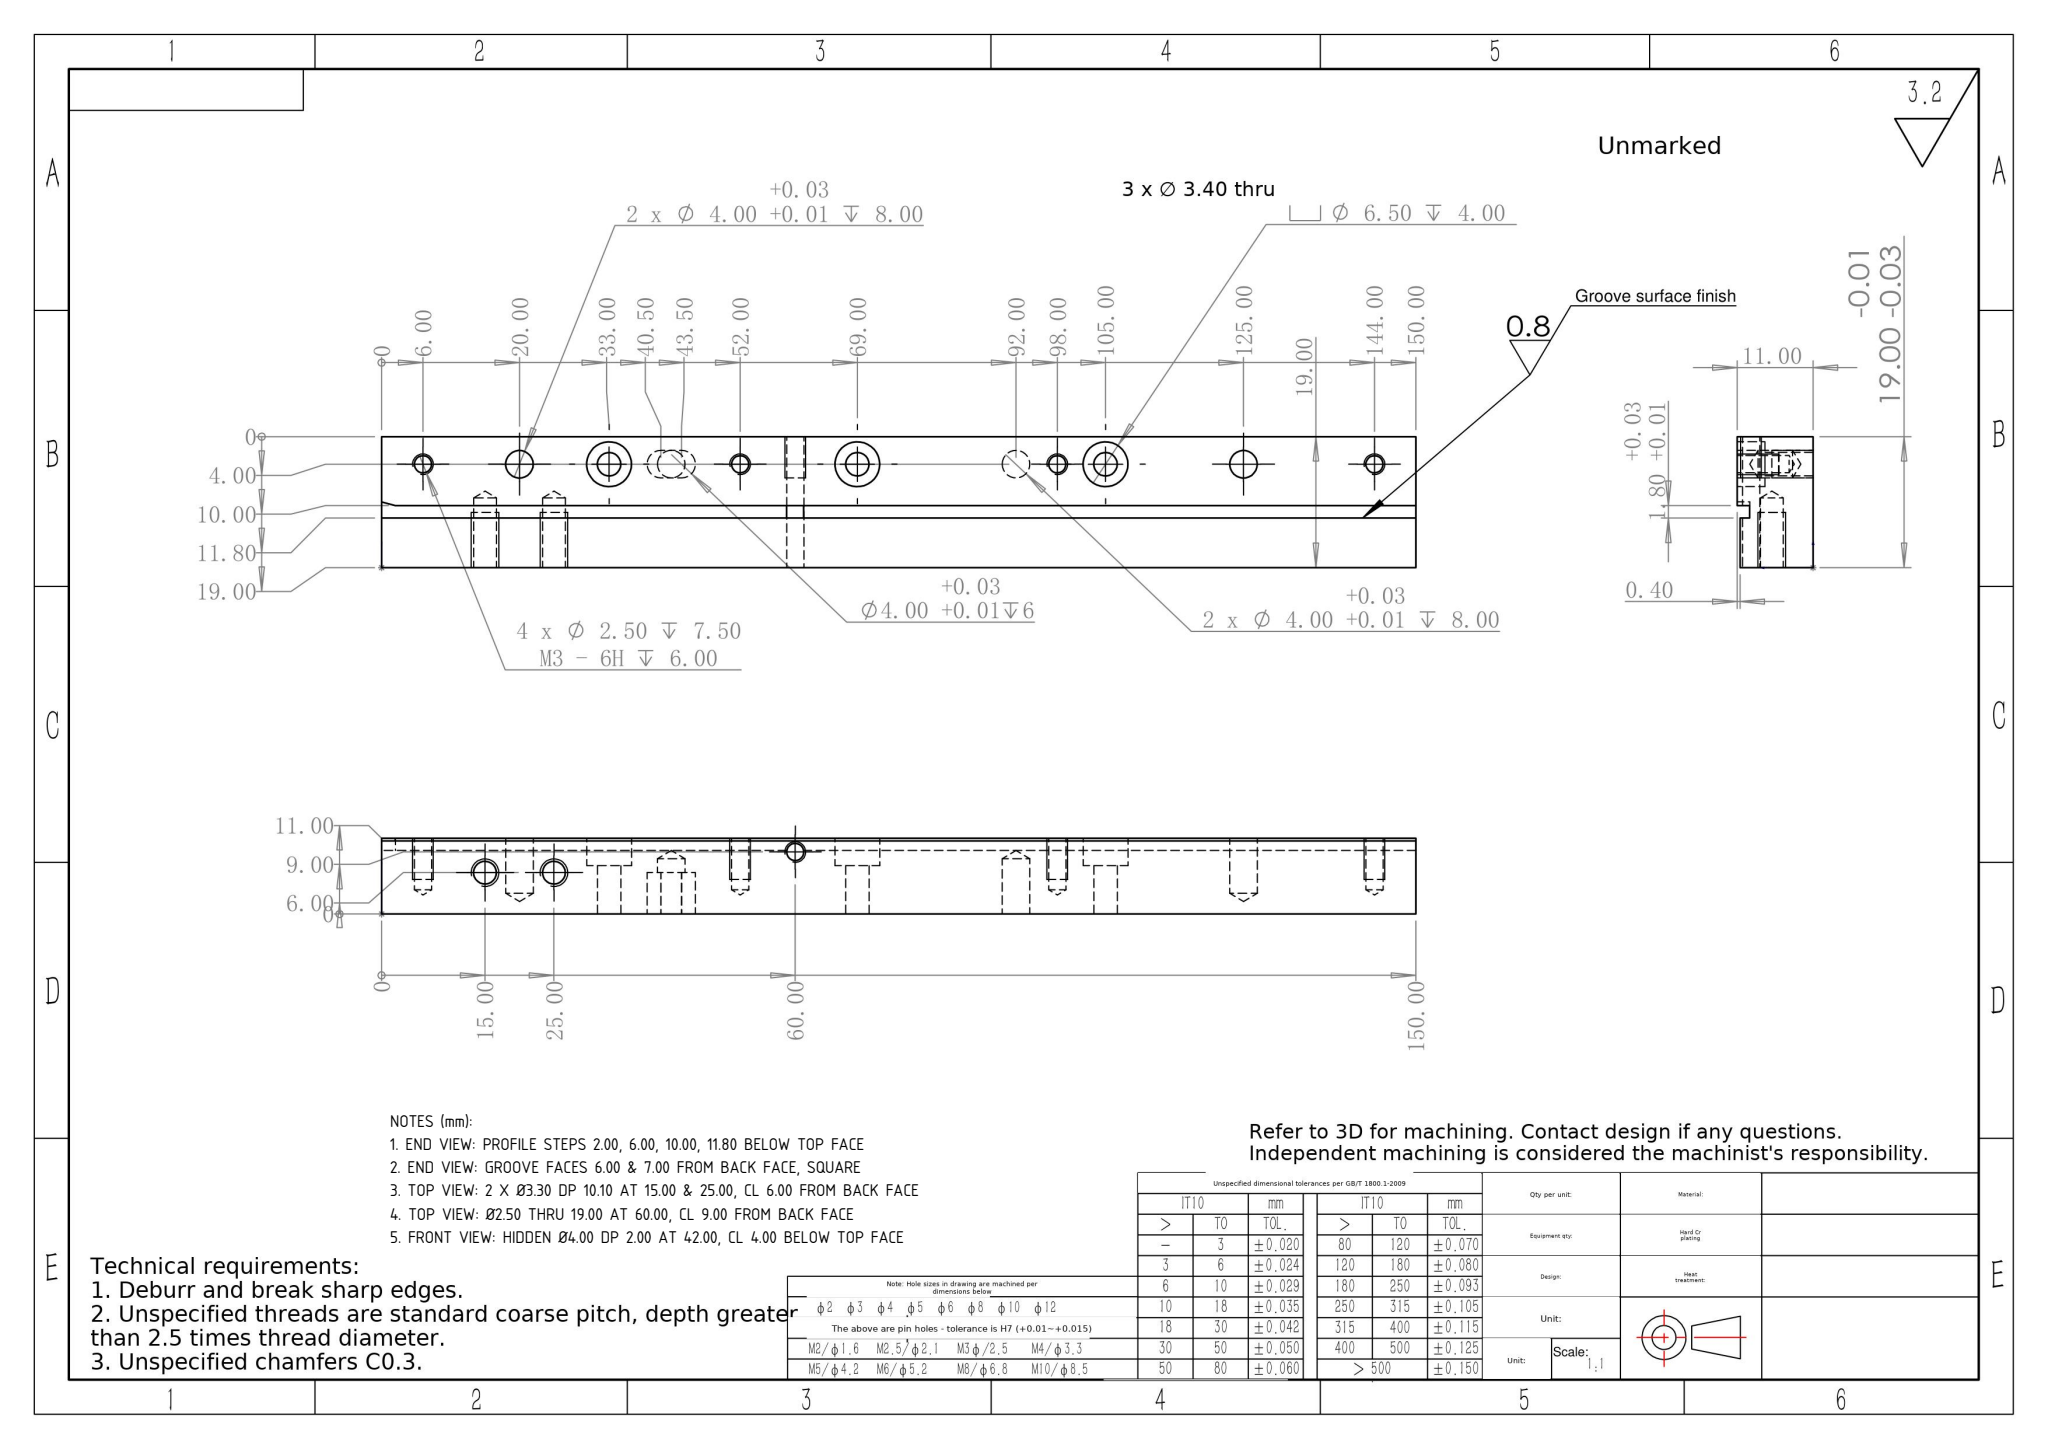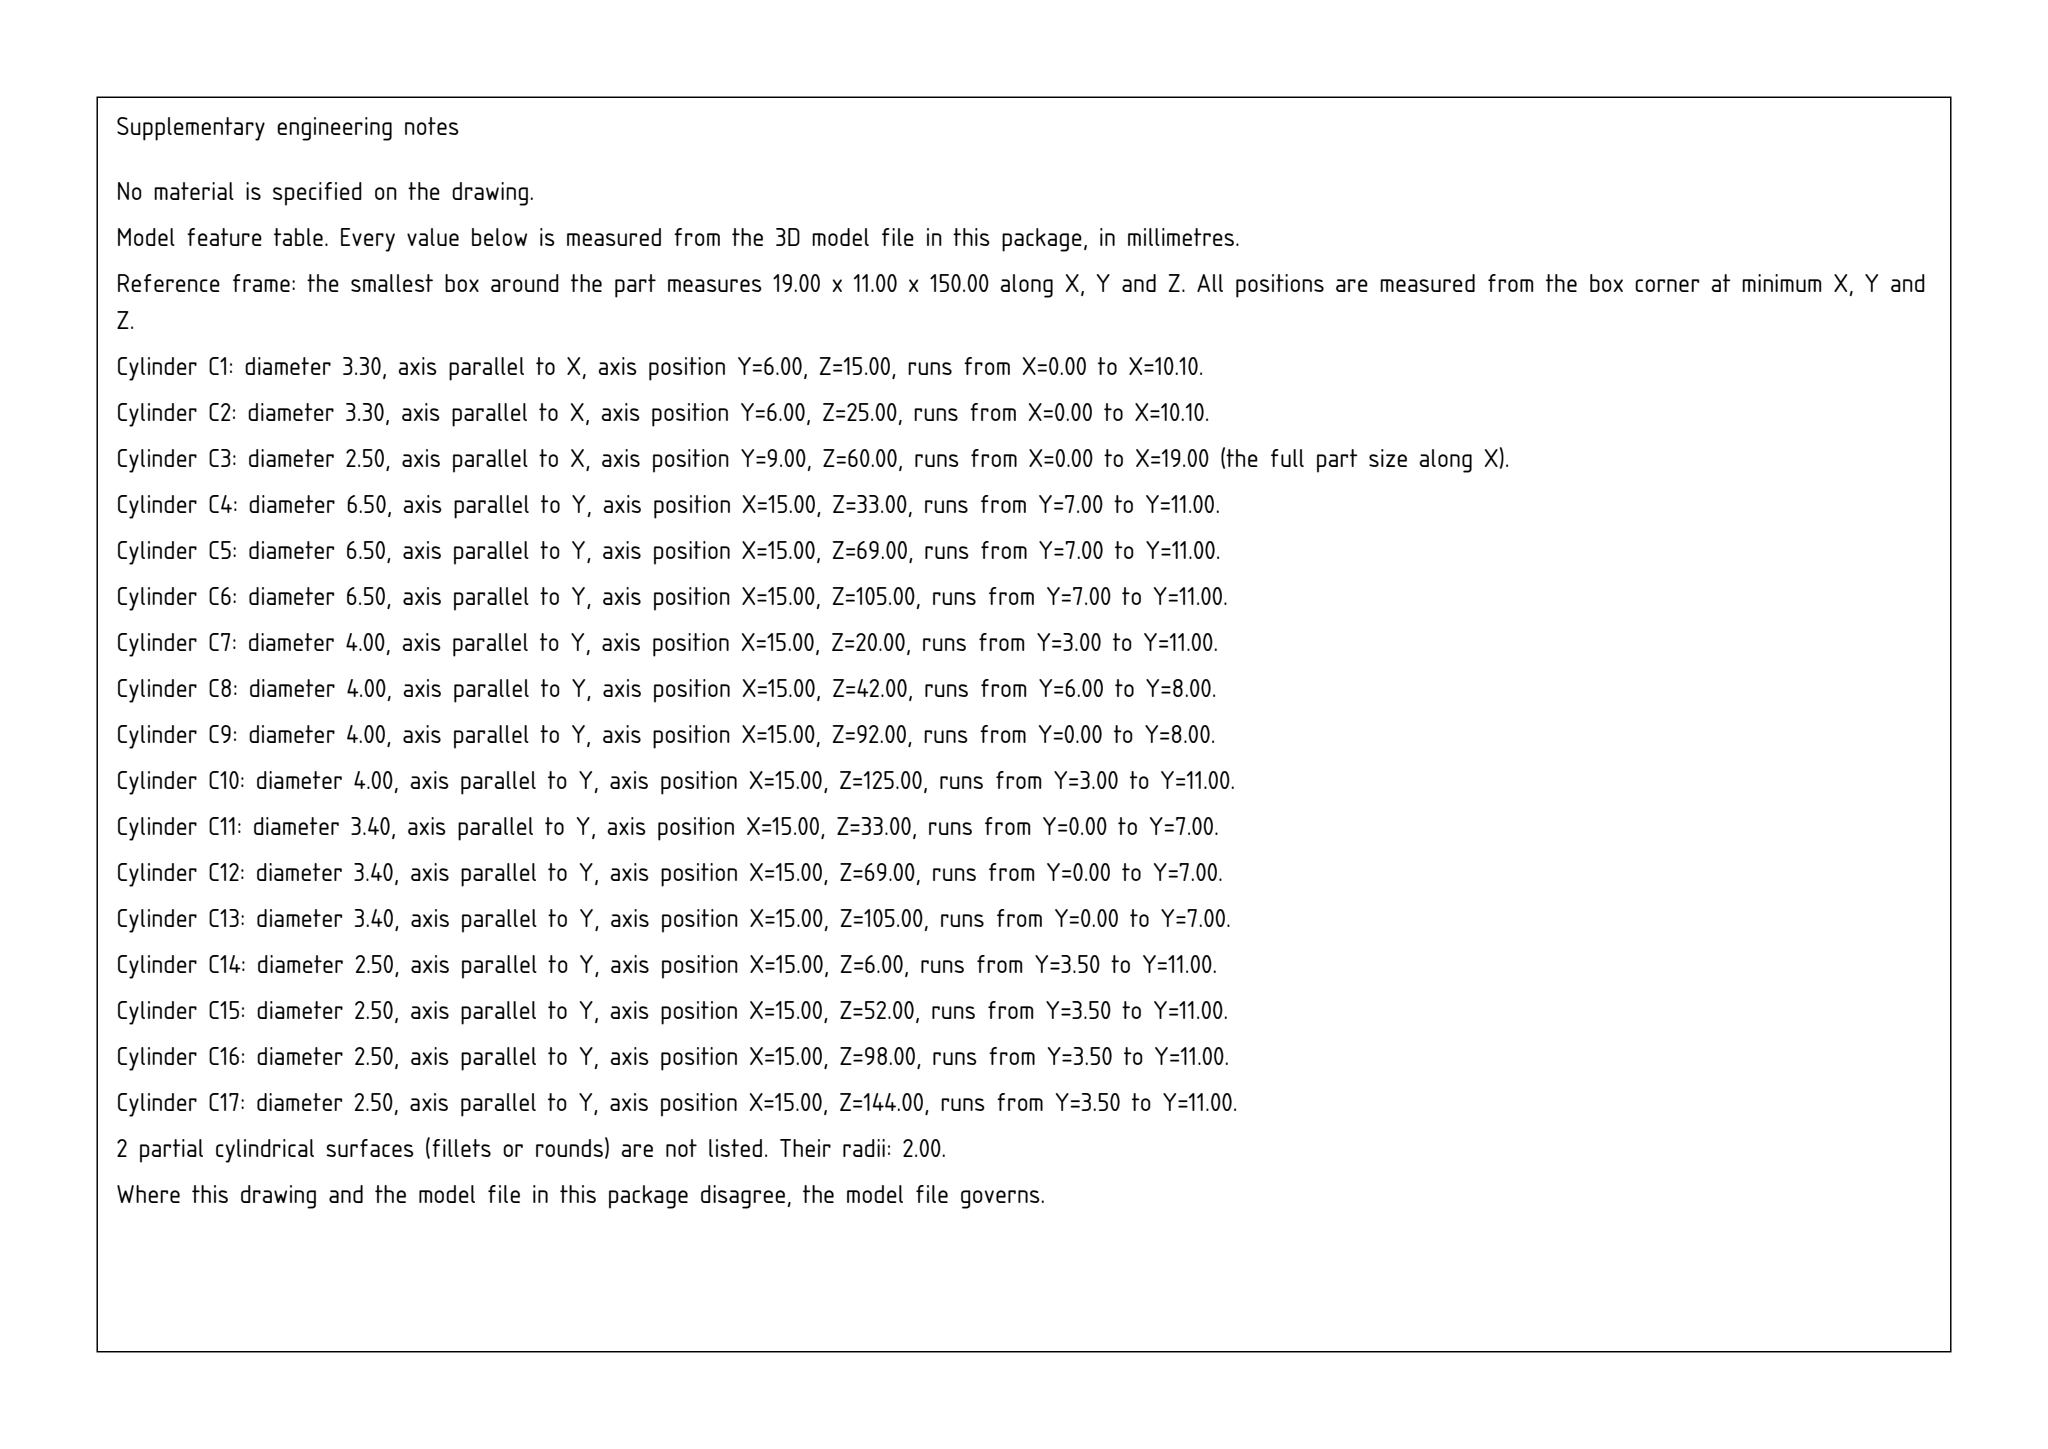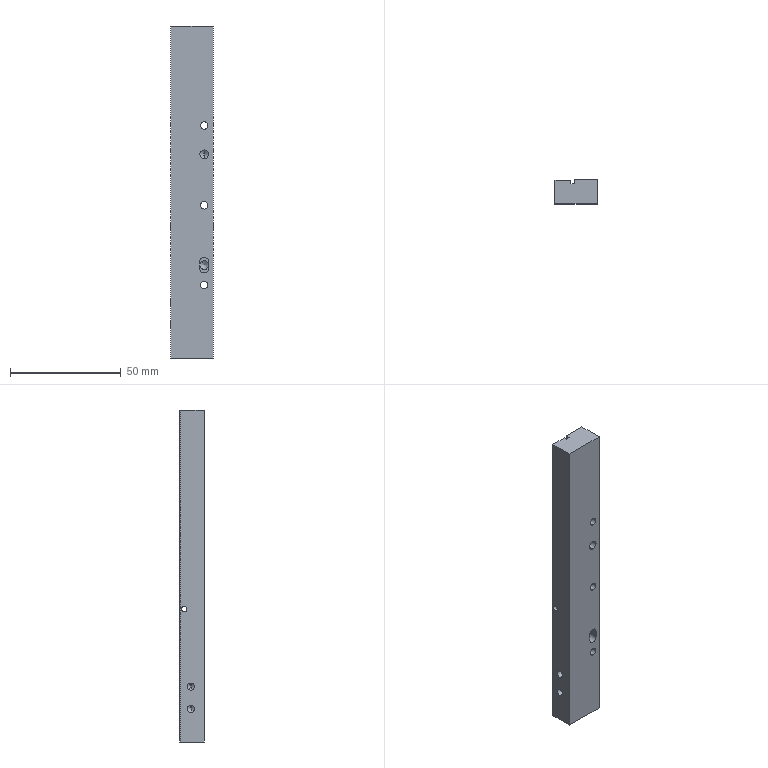Part | SolidWorks | mm | 1 solid | 75 faces | box 19 x 11 x 150 mm | volume 28928 mm3 | cylinder 36 | cone 20 | plane 19 | commonest cylinder face diameters 2.5 x10 4 x10 6.5 x6 3.4 x6 3.3 x4
Drawing notes:
END VIEW: PROFILE STEPS 2.00, 6.00, 10.00, 11.80 BELOW TOP FACE | from the solid: axis_planes x=17.0, 13.0, 9.0, 7.2 vs top face x=19.0 (bbox 19.0)
END VIEW: GROOVE FACES 6.00 & 7.00 FROM BACK FACE, SQUARE | from the solid: axis_planes y=6.0 (x2), y=7.0 (x3); 0.40/1.80 = y10.60/9.20 from front face y=11
TOP VIEW: 2 X Ø3.30 DP 10.10 AT 15.00 & 25.00, CL 6.00 FROM BACK FACE | from the solid: cylinders [3.3,"x",[null,6.0,15.0],10.1] and [3.3,"x",[null,6.0,25.0],10.1]
TOP VIEW: Ø2.50 THRU 19.00 AT 60.00, CL 9.00 FROM BACK FACE | from the solid: cylinder [2.5,"x",[null,9.0,60.0],19.0] = full bbox height 19.0
FRONT VIEW: HIDDEN Ø4.00 DP 2.00 AT 42.00, CL 4.00 BELOW TOP FACE | from the solid: cylinder [4.0,"y",[15.0,null,42.0],2.0]; x=15 is 4.00 below top face x=19
build123d program:
from build123d import *

# Parameters (mm, degrees)
BOSS_EXTRUDE1_DEPTH                             = 150
M3_HEX_SOCKET_HEAD_CAP_SCREW_CBORE1_D           = 3.4
M3_HEX_SOCKET_HEAD_CAP_SCREW_CBORE1_CBORE_D     = 6.5
M3_HEX_SOCKET_HEAD_CAP_SCREW_CBORE1_CBORE_DEPTH = 4
M3_TAPPED_HOLE1_D                               = 2.5
M3_TAPPED_HOLE1_DEPTH                           = 7.5
M3_TAPPED_HOLE1_TIP                             = 0.7511
F_4_0_4_DIAMETER_HOLE1_D                        = 4
F_4_0_4_DIAMETER_HOLE1_DEPTH                    = 8
F_4_0_4_DIAMETER_HOLE1_TIP                      = 1.202
CUT_EXTRUDE1_DEPTH                              = 6
CHAMFER1_SIZE                                   = 2
CHAMFER1_SIZE2                                  = 0.5359
F_4_0_4_DIAMETER_HOLE2_D                        = 4
F_4_0_4_DIAMETER_HOLE2_DEPTH                    = 8
F_4_0_4_DIAMETER_HOLE2_TIP                      = 1.202
M3_TAPPED_HOLE2_D                               = 2.5
M3_TAPPED_HOLE2_DEPTH                           = 20
M3_TAPPED_HOLE2_TIP                             = 0.7511
M4_TAPPED_HOLE1_D                               = 3.3
M4_TAPPED_HOLE1_DEPTH                           = 10.1
M4_TAPPED_HOLE1_TIP                             = 0.9914
SKETCH17_W                                      = 10.048
SKETCH17_H                                      = 6.483
CUT_EXTRUDE2_DEPTH                              = 152.598


with BuildPart() as part:
    # Sketch1 → Boss-Extrude1 (new body)
    with BuildSketch(Plane.XY):
        Polygon((0, 0), (0, 11), (7.2, 11), (7.2, 9.2), (9, 9.2), (9, 11), (19, 11), (19, 0), align=None)
    extrude(amount=BOSS_EXTRUDE1_DEPTH)

    # M3 Hex Socket Head Cap Screw CBORE1 (through all)
    with Locations(Plane(origin=(0, 11, 0), x_dir=(-1, 0, 0), z_dir=(0, 1, 0))):
        with Locations((-15, 105), (-15, 69), (-15, 33)):
            CounterBoreHole(M3_HEX_SOCKET_HEAD_CAP_SCREW_CBORE1_D / 2, M3_HEX_SOCKET_HEAD_CAP_SCREW_CBORE1_CBORE_D / 2, M3_HEX_SOCKET_HEAD_CAP_SCREW_CBORE1_CBORE_DEPTH)

    # M3 Tapped Hole1
    with Locations(Plane(origin=(0, 11, 0), x_dir=(-1, 0, 0), z_dir=(0, 1, 0))):
        with Locations((-15, 144), (-15, 98), (-15, 52), (-15, 6)):
            Hole(M3_TAPPED_HOLE1_D / 2, depth=M3_TAPPED_HOLE1_DEPTH)
            with Locations((0, 0, -(M3_TAPPED_HOLE1_DEPTH + M3_TAPPED_HOLE1_TIP / 2))):  # 118° drill point
                Cone(0, M3_TAPPED_HOLE1_D / 2, M3_TAPPED_HOLE1_TIP, mode=Mode.SUBTRACT)

    # 4.0 _4_ Diameter Hole1
    with Locations(Plane.XZ):
        with Locations((15, 92), (15, 42)):
            Hole(F_4_0_4_DIAMETER_HOLE1_D / 2, depth=F_4_0_4_DIAMETER_HOLE1_DEPTH)
            with Locations((0, 0, -(F_4_0_4_DIAMETER_HOLE1_DEPTH + F_4_0_4_DIAMETER_HOLE1_TIP / 2))):  # 118° drill point
                Cone(0, F_4_0_4_DIAMETER_HOLE1_D / 2, F_4_0_4_DIAMETER_HOLE1_TIP, mode=Mode.SUBTRACT)

    # Sketch8 → Cut-Extrude1 (cut)
    with BuildSketch(Plane.XZ):
        with BuildLine():
            Line((17, 43.5), (17, 40.5))
            ThreePointArc((17, 40.5), (15, 38.5), (13, 40.5))
            Line((13, 40.5), (13, 43.5))
            ThreePointArc((13, 43.5), (15, 45.5), (17, 43.5))
        make_face()
    extrude(amount=-CUT_EXTRUDE1_DEPTH, mode=Mode.SUBTRACT)

    # Chamfer1
    chamfer1_edges = [part.edges().sort_by_distance(p)[0] for p in [
        (9, 10.1, 0),
    ]]
    chamfer1_side = [part.faces().sort_by_distance(p)[0] for p in [
        (9, 10.1, 75),
    ]]
    chamfer(chamfer1_edges, length=CHAMFER1_SIZE, length2=CHAMFER1_SIZE2, reference=chamfer1_side[0])

    # 4.0 _4_ Diameter Hole2
    with Locations(Plane(origin=(0, 11, 0), x_dir=(-1, 0, 0), z_dir=(0, 1, 0))):
        with Locations((-15, 20), (-15, 125)):
            Hole(F_4_0_4_DIAMETER_HOLE2_D / 2, depth=F_4_0_4_DIAMETER_HOLE2_DEPTH)
            with Locations((0, 0, -(F_4_0_4_DIAMETER_HOLE2_DEPTH + F_4_0_4_DIAMETER_HOLE2_TIP / 2))):  # 118° drill point
                Cone(0, F_4_0_4_DIAMETER_HOLE2_D / 2, F_4_0_4_DIAMETER_HOLE2_TIP, mode=Mode.SUBTRACT)

    # M3 Tapped Hole2
    with Locations(Plane(origin=(19, 0, 0), x_dir=(0, 0, -1), z_dir=(1, 0, 0))):
        with Locations((-60, 9)):
            Hole(M3_TAPPED_HOLE2_D / 2, depth=M3_TAPPED_HOLE2_DEPTH)
            with Locations((0, 0, -(M3_TAPPED_HOLE2_DEPTH + M3_TAPPED_HOLE2_TIP / 2))):  # 118° drill point
                Cone(0, M3_TAPPED_HOLE2_D / 2, M3_TAPPED_HOLE2_TIP, mode=Mode.SUBTRACT)

    # M4 Tapped Hole1
    with Locations(Plane.ZY):
        with Locations((15, 6), (25, 6)):
            Hole(M4_TAPPED_HOLE1_D / 2, depth=M4_TAPPED_HOLE1_DEPTH)
            with Locations((0, 0, -(M4_TAPPED_HOLE1_DEPTH + M4_TAPPED_HOLE1_TIP / 2))):  # 118° drill point
                Cone(0, M4_TAPPED_HOLE1_D / 2, M4_TAPPED_HOLE1_TIP, mode=Mode.SUBTRACT)

    # Sketch17 → Cut-Extrude2 (cut, through all)
    with BuildSketch(Plane.XY.offset(150)):
        with Locations((2.906, 13.842)):
            Rectangle(SKETCH17_W, SKETCH17_H)
    extrude(amount=-CUT_EXTRUDE2_DEPTH, mode=Mode.SUBTRACT)


solid = part.part